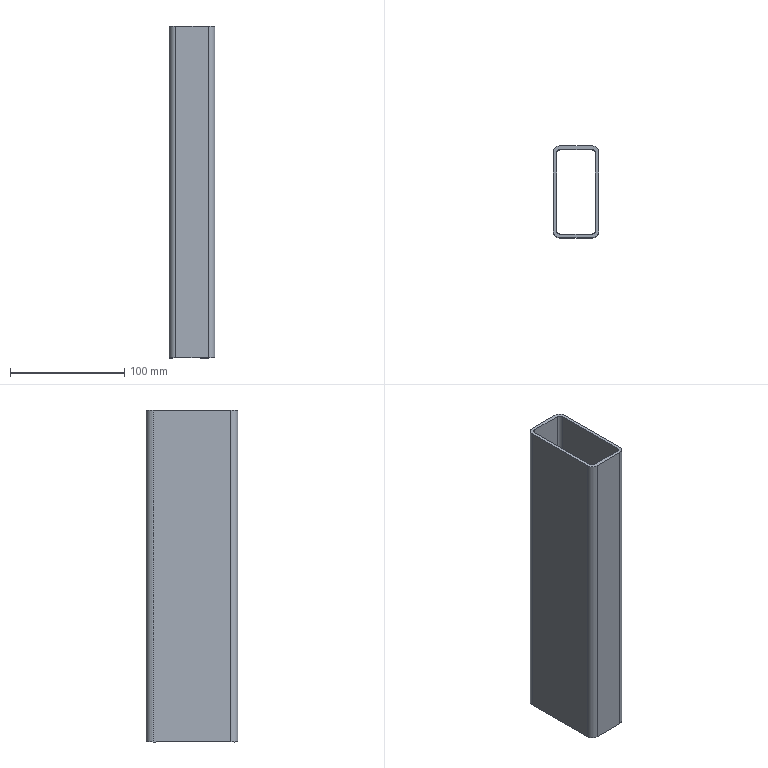Component | SolidWorks | VerticalMovingRectangularTubeWeldment-1_VerticalMovingTube-3 | 1 solid | 18 faces | box 40 x 80 x 290 mm | volume 191639 mm3 | plane 10 | cylinder 8 | commonest cylinder face diameters 12 x4 6 x4 | material Plain Carbon Steel
build123d program:
from build123d import *

# Parameters (mm, degrees)
STRUCTURAL_MEMBER1_DEPTH = 290


with BuildPart() as part:
    # Sketch1 → Structural Member1 (new body)
    with BuildSketch(Plane(origin=(-145, 0, 0), x_dir=(0, 0, -1), z_dir=(1, 0, 0))):
        with BuildLine():
            Line((-14, -40), (14, -40))
            ThreePointArc((14, -40), (18.243, -38.243), (20, -34))
            Line((20, -34), (20, 34))
            ThreePointArc((20, 34), (18.243, 38.243), (14, 40))
            Line((14, 40), (-14, 40))
            ThreePointArc((-14, 40), (-18.243, 38.243), (-20, 34))
            Line((-20, 34), (-20, -34))
            ThreePointArc((-20, -34), (-18.243, -38.243), (-14, -40))
        make_face()
        with BuildLine():
            Line((-14, -37), (14, -37))
            ThreePointArc((14, -37), (16.121, -36.121), (17, -34))
            Line((17, -34), (17, 34))
            ThreePointArc((17, 34), (16.121, 36.121), (14, 37))
            Line((14, 37), (-14, 37))
            ThreePointArc((-14, 37), (-16.121, 36.121), (-17, 34))
            Line((-17, 34), (-17, -34))
            ThreePointArc((-17, -34), (-16.121, -36.121), (-14, -37))
        make_face(mode=Mode.SUBTRACT)
    extrude(amount=STRUCTURAL_MEMBER1_DEPTH)


solid = part.part

# Placed as in the assembly
solid = solid.moved(Location((250, 0, 165), (0, 90, 0)))
STEP:
#1=COLOUR_RGB('',0.7922,0.8196,0.9333);
#2=FILL_AREA_STYLE_COLOUR('',#1);
#3=FILL_AREA_STYLE('',(#2));
#4=SURFACE_STYLE_FILL_AREA(#3);
#5=SURFACE_SIDE_STYLE('',(#4));
#6=SURFACE_STYLE_USAGE(.BOTH.,#5);
#7=PRESENTATION_STYLE_ASSIGNMENT((#6));
#8=CARTESIAN_POINT('',(10.63,1.339,0.7874));
#9=VERTEX_POINT('',#8);
#10=CARTESIAN_POINT('',(10.394,1.575,0.7874));
#11=VERTEX_POINT('',#10);
#12=CARTESIAN_POINT('',(10.394,1.339,0.7874));
#13=DIRECTION('',(-0.,0.,1.));
#14=DIRECTION('',(1.,0.,0.));
#15=AXIS2_PLACEMENT_3D('',#12,#13,#14);
#16=CIRCLE('',#15,0.2362);
#17=EDGE_CURVE('',#9,#11,#16,.T.);
#18=ORIENTED_EDGE('',*,*,#17,.T.);
#19=CARTESIAN_POINT('',(10.394,1.575,12.205));
#20=VERTEX_POINT('',#19);
#21=CARTESIAN_POINT('',(10.394,1.575,12.205));
#22=DIRECTION('',(0.,0.,-1.));
#23=VECTOR('',#22,39.37);
#24=LINE('',#21,#23);
#25=EDGE_CURVE('',#20,#11,#24,.T.);
#26=ORIENTED_EDGE('',*,*,#25,.F.);
#27=CARTESIAN_POINT('',(10.63,1.339,12.205));
#28=VERTEX_POINT('',#27);
#29=CARTESIAN_POINT('',(10.394,1.339,12.205));
#30=DIRECTION('',(-0.,0.,1.));
#31=DIRECTION('',(1.,0.,0.));
#32=AXIS2_PLACEMENT_3D('',#29,#30,#31);
#33=CIRCLE('',#32,0.2362);
#34=EDGE_CURVE('',#28,#20,#33,.T.);
#35=ORIENTED_EDGE('',*,*,#34,.F.);
#36=CARTESIAN_POINT('',(10.63,1.339,12.205));
#37=DIRECTION('',(0.,0.,-1.));
#38=VECTOR('',#37,39.37);
#39=LINE('',#36,#38);
#40=EDGE_CURVE('',#28,#9,#39,.T.);
#41=ORIENTED_EDGE('',*,*,#40,.T.);
#42=EDGE_LOOP('',(#18,#26,#35,#41));
#43=FACE_OUTER_BOUND('',#42,.T.);
#44=CARTESIAN_POINT('',(10.394,1.339,12.205));
#45=DIRECTION('',(0.,0.,-1.));
#46=DIRECTION('',(-1.,0.,0.));
#47=AXIS2_PLACEMENT_3D('',#44,#45,#46);
#48=CYLINDRICAL_SURFACE('',#47,0.2362);
#49=ADVANCED_FACE('',(#43),#48,.T.);
#50=CARTESIAN_POINT('',(9.291,1.575,0.7874));
#51=VERTEX_POINT('',#50);
#52=CARTESIAN_POINT('',(10.394,1.575,0.7874));
#53=DIRECTION('',(-1.,0.,0.));
#54=VECTOR('',#53,39.37);
#55=LINE('',#52,#54);
#56=EDGE_CURVE('',#11,#51,#55,.T.);
#57=ORIENTED_EDGE('',*,*,#56,.T.);
#58=CARTESIAN_POINT('',(9.291,1.575,12.205));
#59=VERTEX_POINT('',#58);
#60=CARTESIAN_POINT('',(9.291,1.575,12.205));
#61=DIRECTION('',(0.,0.,-1.));
#62=VECTOR('',#61,39.37);
#63=LINE('',#60,#62);
#64=EDGE_CURVE('',#59,#51,#63,.T.);
#65=ORIENTED_EDGE('',*,*,#64,.F.);
#66=CARTESIAN_POINT('',(10.394,1.575,12.205));
#67=DIRECTION('',(-1.,0.,0.));
#68=VECTOR('',#67,39.37);
#69=LINE('',#66,#68);
#70=EDGE_CURVE('',#20,#59,#69,.T.);
#71=ORIENTED_EDGE('',*,*,#70,.F.);
#72=ORIENTED_EDGE('',*,*,#25,.T.);
#73=EDGE_LOOP('',(#57,#65,#71,#72));
#74=FACE_OUTER_BOUND('',#73,.T.);
#75=CARTESIAN_POINT('',(10.394,1.575,12.205));
#76=DIRECTION('',(-0.,-1.,0.));
#77=DIRECTION('',(1.,-0.,-0.));
#78=AXIS2_PLACEMENT_3D('',#75,#76,#77);
#79=PLANE('',#78);
#80=ADVANCED_FACE('',(#74),#79,.F.);
#81=CARTESIAN_POINT('',(9.055,1.339,0.7874));
#82=VERTEX_POINT('',#81);
#83=CARTESIAN_POINT('',(9.291,1.339,0.7874));
#84=DIRECTION('',(-0.,0.,1.));
#85=DIRECTION('',(1.,0.,0.));
#86=AXIS2_PLACEMENT_3D('',#83,#84,#85);
#87=CIRCLE('',#86,0.2362);
#88=EDGE_CURVE('',#51,#82,#87,.T.);
#89=ORIENTED_EDGE('',*,*,#88,.T.);
#90=CARTESIAN_POINT('',(9.055,1.339,12.205));
#91=VERTEX_POINT('',#90);
#92=CARTESIAN_POINT('',(9.055,1.339,12.205));
#93=DIRECTION('',(0.,0.,-1.));
#94=VECTOR('',#93,39.37);
#95=LINE('',#92,#94);
#96=EDGE_CURVE('',#91,#82,#95,.T.);
#97=ORIENTED_EDGE('',*,*,#96,.F.);
#98=CARTESIAN_POINT('',(9.291,1.339,12.205));
#99=DIRECTION('',(-0.,0.,1.));
#100=DIRECTION('',(1.,0.,0.));
#101=AXIS2_PLACEMENT_3D('',#98,#99,#100);
#102=CIRCLE('',#101,0.2362);
#103=EDGE_CURVE('',#59,#91,#102,.T.);
#104=ORIENTED_EDGE('',*,*,#103,.F.);
#105=ORIENTED_EDGE('',*,*,#64,.T.);
#106=EDGE_LOOP('',(#89,#97,#104,#105));
#107=FACE_OUTER_BOUND('',#106,.T.);
#108=CARTESIAN_POINT('',(9.291,1.339,12.205));
#109=DIRECTION('',(0.,0.,-1.));
#110=DIRECTION('',(-1.,0.,0.));
#111=AXIS2_PLACEMENT_3D('',#108,#109,#110);
#112=CYLINDRICAL_SURFACE('',#111,0.2362);
#113=ADVANCED_FACE('',(#107),#112,.T.);
#114=CARTESIAN_POINT('',(9.055,-1.339,0.7874));
#115=VERTEX_POINT('',#114);
#116=CARTESIAN_POINT('',(9.055,-1.339,0.7874));
#117=DIRECTION('',(0.,-1.,0.));
#118=VECTOR('',#117,39.37);
#119=LINE('',#116,#118);
#120=EDGE_CURVE('',#82,#115,#119,.T.);
#121=ORIENTED_EDGE('',*,*,#120,.T.);
#122=CARTESIAN_POINT('',(9.055,-1.339,12.205));
#123=VERTEX_POINT('',#122);
#124=CARTESIAN_POINT('',(9.055,-1.339,12.205));
#125=DIRECTION('',(0.,0.,-1.));
#126=VECTOR('',#125,39.37);
#127=LINE('',#124,#126);
#128=EDGE_CURVE('',#123,#115,#127,.T.);
#129=ORIENTED_EDGE('',*,*,#128,.F.);
#130=CARTESIAN_POINT('',(9.055,-1.339,12.205));
#131=DIRECTION('',(0.,-1.,0.));
#132=VECTOR('',#131,39.37);
#133=LINE('',#130,#132);
#134=EDGE_CURVE('',#91,#123,#133,.T.);
#135=ORIENTED_EDGE('',*,*,#134,.F.);
#136=ORIENTED_EDGE('',*,*,#96,.T.);
#137=EDGE_LOOP('',(#121,#129,#135,#136));
#138=FACE_OUTER_BOUND('',#137,.T.);
#139=CARTESIAN_POINT('',(9.055,-1.339,12.205));
#140=DIRECTION('',(1.,-0.,0.));
#141=DIRECTION('',(0.,0.,-1.));
#142=AXIS2_PLACEMENT_3D('',#139,#140,#141);
#143=PLANE('',#142);
#144=ADVANCED_FACE('',(#138),#143,.F.);
#145=CARTESIAN_POINT('',(9.291,-1.575,0.7874));
#146=VERTEX_POINT('',#145);
#147=CARTESIAN_POINT('',(9.291,-1.339,0.7874));
#148=DIRECTION('',(-0.,0.,1.));
#149=DIRECTION('',(1.,0.,0.));
#150=AXIS2_PLACEMENT_3D('',#147,#148,#149);
#151=CIRCLE('',#150,0.2362);
#152=EDGE_CURVE('',#115,#146,#151,.T.);
#153=ORIENTED_EDGE('',*,*,#152,.T.);
#154=CARTESIAN_POINT('',(9.291,-1.575,12.205));
#155=VERTEX_POINT('',#154);
#156=CARTESIAN_POINT('',(9.291,-1.575,12.205));
#157=DIRECTION('',(0.,0.,-1.));
#158=VECTOR('',#157,39.37);
#159=LINE('',#156,#158);
#160=EDGE_CURVE('',#155,#146,#159,.T.);
#161=ORIENTED_EDGE('',*,*,#160,.F.);
#162=CARTESIAN_POINT('',(9.291,-1.339,12.205));
#163=DIRECTION('',(-0.,0.,1.));
#164=DIRECTION('',(1.,0.,0.));
#165=AXIS2_PLACEMENT_3D('',#162,#163,#164);
#166=CIRCLE('',#165,0.2362);
#167=EDGE_CURVE('',#123,#155,#166,.T.);
#168=ORIENTED_EDGE('',*,*,#167,.F.);
#169=ORIENTED_EDGE('',*,*,#128,.T.);
#170=EDGE_LOOP('',(#153,#161,#168,#169));
#171=FACE_OUTER_BOUND('',#170,.T.);
#172=CARTESIAN_POINT('',(9.291,-1.339,12.205));
#173=DIRECTION('',(0.,0.,-1.));
#174=DIRECTION('',(-1.,0.,0.));
#175=AXIS2_PLACEMENT_3D('',#172,#173,#174);
#176=CYLINDRICAL_SURFACE('',#175,0.2362);
#177=ADVANCED_FACE('',(#171),#176,.T.);
#178=CARTESIAN_POINT('',(10.394,-1.575,0.7874));
#179=VERTEX_POINT('',#178);
#180=CARTESIAN_POINT('',(9.291,-1.575,0.7874));
#181=DIRECTION('',(1.,-0.,-0.));
#182=VECTOR('',#181,39.37);
#183=LINE('',#180,#182);
#184=EDGE_CURVE('',#146,#179,#183,.T.);
#185=ORIENTED_EDGE('',*,*,#184,.T.);
#186=CARTESIAN_POINT('',(10.394,-1.575,12.205));
#187=VERTEX_POINT('',#186);
#188=CARTESIAN_POINT('',(10.394,-1.575,12.205));
#189=DIRECTION('',(0.,0.,-1.));
#190=VECTOR('',#189,39.37);
#191=LINE('',#188,#190);
#192=EDGE_CURVE('',#187,#179,#191,.T.);
#193=ORIENTED_EDGE('',*,*,#192,.F.);
#194=CARTESIAN_POINT('',(9.291,-1.575,12.205));
#195=DIRECTION('',(1.,-0.,-0.));
#196=VECTOR('',#195,39.37);
#197=LINE('',#194,#196);
#198=EDGE_CURVE('',#155,#187,#197,.T.);
#199=ORIENTED_EDGE('',*,*,#198,.F.);
#200=ORIENTED_EDGE('',*,*,#160,.T.);
#201=EDGE_LOOP('',(#185,#193,#199,#200));
#202=FACE_OUTER_BOUND('',#201,.T.);
#203=CARTESIAN_POINT('',(9.291,-1.575,12.205));
#204=DIRECTION('',(0.,1.,-0.));
#205=DIRECTION('',(-1.,0.,0.));
#206=AXIS2_PLACEMENT_3D('',#203,#204,#205);
#207=PLANE('',#206);
#208=ADVANCED_FACE('',(#202),#207,.F.);
#209=CARTESIAN_POINT('',(10.63,-1.339,0.7874));
#210=VERTEX_POINT('',#209);
#211=CARTESIAN_POINT('',(10.394,-1.339,0.7874));
#212=DIRECTION('',(-0.,0.,1.));
#213=DIRECTION('',(1.,0.,0.));
#214=AXIS2_PLACEMENT_3D('',#211,#212,#213);
#215=CIRCLE('',#214,0.2362);
#216=EDGE_CURVE('',#179,#210,#215,.T.);
#217=ORIENTED_EDGE('',*,*,#216,.T.);
#218=CARTESIAN_POINT('',(10.63,-1.339,12.205));
#219=VERTEX_POINT('',#218);
#220=CARTESIAN_POINT('',(10.63,-1.339,12.205));
#221=DIRECTION('',(0.,0.,-1.));
#222=VECTOR('',#221,39.37);
#223=LINE('',#220,#222);
#224=EDGE_CURVE('',#219,#210,#223,.T.);
#225=ORIENTED_EDGE('',*,*,#224,.F.);
#226=CARTESIAN_POINT('',(10.394,-1.339,12.205));
#227=DIRECTION('',(-0.,0.,1.));
#228=DIRECTION('',(1.,0.,0.));
#229=AXIS2_PLACEMENT_3D('',#226,#227,#228);
#230=CIRCLE('',#229,0.2362);
#231=EDGE_CURVE('',#187,#219,#230,.T.);
#232=ORIENTED_EDGE('',*,*,#231,.F.);
#233=ORIENTED_EDGE('',*,*,#192,.T.);
#234=EDGE_LOOP('',(#217,#225,#232,#233));
#235=FACE_OUTER_BOUND('',#234,.T.);
#236=CARTESIAN_POINT('',(10.394,-1.339,12.205));
#237=DIRECTION('',(0.,0.,-1.));
#238=DIRECTION('',(-1.,0.,0.));
#239=AXIS2_PLACEMENT_3D('',#236,#237,#238);
#240=CYLINDRICAL_SURFACE('',#239,0.2362);
#241=ADVANCED_FACE('',(#235),#240,.T.);
#242=CARTESIAN_POINT('',(9.291,1.457,0.7874));
#243=VERTEX_POINT('',#242);
#244=CARTESIAN_POINT('',(9.173,1.339,0.7874));
#245=VERTEX_POINT('',#244);
#246=CARTESIAN_POINT('',(9.291,1.339,0.7874));
#247=DIRECTION('',(-0.,0.,1.));
#248=DIRECTION('',(1.,0.,0.));
#249=AXIS2_PLACEMENT_3D('',#246,#247,#248);
#250=CIRCLE('',#249,0.1181);
#251=EDGE_CURVE('',#243,#245,#250,.T.);
#252=ORIENTED_EDGE('',*,*,#251,.F.);
#253=CARTESIAN_POINT('',(9.291,1.457,12.205));
#254=VERTEX_POINT('',#253);
#255=CARTESIAN_POINT('',(9.291,1.457,12.205));
#256=DIRECTION('',(0.,0.,-1.));
#257=VECTOR('',#256,39.37);
#258=LINE('',#255,#257);
#259=EDGE_CURVE('',#254,#243,#258,.T.);
#260=ORIENTED_EDGE('',*,*,#259,.F.);
#261=CARTESIAN_POINT('',(9.173,1.339,12.205));
#262=VERTEX_POINT('',#261);
#263=CARTESIAN_POINT('',(9.291,1.339,12.205));
#264=DIRECTION('',(-0.,0.,1.));
#265=DIRECTION('',(1.,0.,0.));
#266=AXIS2_PLACEMENT_3D('',#263,#264,#265);
#267=CIRCLE('',#266,0.1181);
#268=EDGE_CURVE('',#254,#262,#267,.T.);
#269=ORIENTED_EDGE('',*,*,#268,.T.);
#270=CARTESIAN_POINT('',(9.173,1.339,12.205));
#271=DIRECTION('',(0.,0.,-1.));
#272=VECTOR('',#271,39.37);
#273=LINE('',#270,#272);
#274=EDGE_CURVE('',#262,#245,#273,.T.);
#275=ORIENTED_EDGE('',*,*,#274,.T.);
#276=EDGE_LOOP('',(#252,#260,#269,#275));
#277=FACE_OUTER_BOUND('',#276,.T.);
#278=CARTESIAN_POINT('',(9.291,1.339,12.205));
#279=DIRECTION('',(0.,0.,-1.));
#280=DIRECTION('',(-1.,0.,0.));
#281=AXIS2_PLACEMENT_3D('',#278,#279,#280);
#282=CYLINDRICAL_SURFACE('',#281,0.1181);
#283=ADVANCED_FACE('',(#277),#282,.F.);
#284=CARTESIAN_POINT('',(10.394,1.457,0.7874));
#285=VERTEX_POINT('',#284);
#286=CARTESIAN_POINT('',(10.394,1.457,0.7874));
#287=DIRECTION('',(-1.,0.,0.));
#288=VECTOR('',#287,39.37);
#289=LINE('',#286,#288);
#290=EDGE_CURVE('',#285,#243,#289,.T.);
#291=ORIENTED_EDGE('',*,*,#290,.F.);
#292=CARTESIAN_POINT('',(10.394,1.457,12.205));
#293=VERTEX_POINT('',#292);
#294=CARTESIAN_POINT('',(10.394,1.457,12.205));
#295=DIRECTION('',(0.,0.,-1.));
#296=VECTOR('',#295,39.37);
#297=LINE('',#294,#296);
#298=EDGE_CURVE('',#293,#285,#297,.T.);
#299=ORIENTED_EDGE('',*,*,#298,.F.);
#300=CARTESIAN_POINT('',(10.394,1.457,12.205));
#301=DIRECTION('',(-1.,0.,0.));
#302=VECTOR('',#301,39.37);
#303=LINE('',#300,#302);
#304=EDGE_CURVE('',#293,#254,#303,.T.);
#305=ORIENTED_EDGE('',*,*,#304,.T.);
#306=ORIENTED_EDGE('',*,*,#259,.T.);
#307=EDGE_LOOP('',(#291,#299,#305,#306));
#308=FACE_OUTER_BOUND('',#307,.T.);
#309=CARTESIAN_POINT('',(10.394,1.457,12.205));
#310=DIRECTION('',(-0.,-1.,0.));
#311=DIRECTION('',(1.,-0.,-0.));
#312=AXIS2_PLACEMENT_3D('',#309,#310,#311);
#313=PLANE('',#312);
#314=ADVANCED_FACE('',(#308),#313,.T.);
#315=CARTESIAN_POINT('',(10.512,1.339,0.7874));
#316=VERTEX_POINT('',#315);
#317=CARTESIAN_POINT('',(10.394,1.339,0.7874));
#318=DIRECTION('',(-0.,0.,1.));
#319=DIRECTION('',(1.,0.,0.));
#320=AXIS2_PLACEMENT_3D('',#317,#318,#319);
#321=CIRCLE('',#320,0.1181);
#322=EDGE_CURVE('',#316,#285,#321,.T.);
#323=ORIENTED_EDGE('',*,*,#322,.F.);
#324=CARTESIAN_POINT('',(10.512,1.339,12.205));
#325=VERTEX_POINT('',#324);
#326=CARTESIAN_POINT('',(10.512,1.339,12.205));
#327=DIRECTION('',(0.,0.,-1.));
#328=VECTOR('',#327,39.37);
#329=LINE('',#326,#328);
#330=EDGE_CURVE('',#325,#316,#329,.T.);
#331=ORIENTED_EDGE('',*,*,#330,.F.);
#332=CARTESIAN_POINT('',(10.394,1.339,12.205));
#333=DIRECTION('',(-0.,0.,1.));
#334=DIRECTION('',(1.,0.,0.));
#335=AXIS2_PLACEMENT_3D('',#332,#333,#334);
#336=CIRCLE('',#335,0.1181);
#337=EDGE_CURVE('',#325,#293,#336,.T.);
#338=ORIENTED_EDGE('',*,*,#337,.T.);
#339=ORIENTED_EDGE('',*,*,#298,.T.);
#340=EDGE_LOOP('',(#323,#331,#338,#339));
#341=FACE_OUTER_BOUND('',#340,.T.);
#342=CARTESIAN_POINT('',(10.394,1.339,12.205));
#343=DIRECTION('',(0.,0.,-1.));
#344=DIRECTION('',(-1.,0.,0.));
#345=AXIS2_PLACEMENT_3D('',#342,#343,#344);
#346=CYLINDRICAL_SURFACE('',#345,0.1181);
#347=ADVANCED_FACE('',(#341),#346,.F.);
#348=CARTESIAN_POINT('',(10.512,-1.339,0.7874));
#349=VERTEX_POINT('',#348);
#350=CARTESIAN_POINT('',(10.512,1.339,0.7874));
#351=DIRECTION('',(-0.,1.,0.));
#352=VECTOR('',#351,39.37);
#353=LINE('',#350,#352);
#354=EDGE_CURVE('',#349,#316,#353,.T.);
#355=ORIENTED_EDGE('',*,*,#354,.F.);
#356=CARTESIAN_POINT('',(10.512,-1.339,12.205));
#357=VERTEX_POINT('',#356);
#358=CARTESIAN_POINT('',(10.512,-1.339,12.205));
#359=DIRECTION('',(0.,0.,-1.));
#360=VECTOR('',#359,39.37);
#361=LINE('',#358,#360);
#362=EDGE_CURVE('',#357,#349,#361,.T.);
#363=ORIENTED_EDGE('',*,*,#362,.F.);
#364=CARTESIAN_POINT('',(10.512,1.339,12.205));
#365=DIRECTION('',(-0.,1.,0.));
#366=VECTOR('',#365,39.37);
#367=LINE('',#364,#366);
#368=EDGE_CURVE('',#357,#325,#367,.T.);
#369=ORIENTED_EDGE('',*,*,#368,.T.);
#370=ORIENTED_EDGE('',*,*,#330,.T.);
#371=EDGE_LOOP('',(#355,#363,#369,#370));
#372=FACE_OUTER_BOUND('',#371,.T.);
#373=CARTESIAN_POINT('',(10.512,1.339,12.205));
#374=DIRECTION('',(-1.,0.,-0.));
#375=DIRECTION('',(-0.,0.,1.));
#376=AXIS2_PLACEMENT_3D('',#373,#374,#375);
#377=PLANE('',#376);
#378=ADVANCED_FACE('',(#372),#377,.T.);
#379=CARTESIAN_POINT('',(10.394,-1.457,0.7874));
#380=VERTEX_POINT('',#379);
#381=CARTESIAN_POINT('',(10.394,-1.339,0.7874));
#382=DIRECTION('',(-0.,0.,1.));
#383=DIRECTION('',(1.,0.,0.));
#384=AXIS2_PLACEMENT_3D('',#381,#382,#383);
#385=CIRCLE('',#384,0.1181);
#386=EDGE_CURVE('',#380,#349,#385,.T.);
#387=ORIENTED_EDGE('',*,*,#386,.F.);
#388=CARTESIAN_POINT('',(10.394,-1.457,12.205));
#389=VERTEX_POINT('',#388);
#390=CARTESIAN_POINT('',(10.394,-1.457,12.205));
#391=DIRECTION('',(0.,0.,-1.));
#392=VECTOR('',#391,39.37);
#393=LINE('',#390,#392);
#394=EDGE_CURVE('',#389,#380,#393,.T.);
#395=ORIENTED_EDGE('',*,*,#394,.F.);
#396=CARTESIAN_POINT('',(10.394,-1.339,12.205));
#397=DIRECTION('',(-0.,0.,1.));
#398=DIRECTION('',(1.,0.,0.));
#399=AXIS2_PLACEMENT_3D('',#396,#397,#398);
#400=CIRCLE('',#399,0.1181);
#401=EDGE_CURVE('',#389,#357,#400,.T.);
#402=ORIENTED_EDGE('',*,*,#401,.T.);
#403=ORIENTED_EDGE('',*,*,#362,.T.);
#404=EDGE_LOOP('',(#387,#395,#402,#403));
#405=FACE_OUTER_BOUND('',#404,.T.);
#406=CARTESIAN_POINT('',(10.394,-1.339,12.205));
#407=DIRECTION('',(0.,0.,-1.));
#408=DIRECTION('',(-1.,0.,0.));
#409=AXIS2_PLACEMENT_3D('',#406,#407,#408);
#410=CYLINDRICAL_SURFACE('',#409,0.1181);
#411=ADVANCED_FACE('',(#405),#410,.F.);
#412=CARTESIAN_POINT('',(9.291,-1.457,0.7874));
#413=VERTEX_POINT('',#412);
#414=CARTESIAN_POINT('',(9.291,-1.457,0.7874));
#415=DIRECTION('',(1.,-0.,-0.));
#416=VECTOR('',#415,39.37);
#417=LINE('',#414,#416);
#418=EDGE_CURVE('',#413,#380,#417,.T.);
#419=ORIENTED_EDGE('',*,*,#418,.F.);
#420=CARTESIAN_POINT('',(9.291,-1.457,12.205));
#421=VERTEX_POINT('',#420);
#422=CARTESIAN_POINT('',(9.291,-1.457,12.205));
#423=DIRECTION('',(0.,0.,-1.));
#424=VECTOR('',#423,39.37);
#425=LINE('',#422,#424);
#426=EDGE_CURVE('',#421,#413,#425,.T.);
#427=ORIENTED_EDGE('',*,*,#426,.F.);
#428=CARTESIAN_POINT('',(9.291,-1.457,12.205));
#429=DIRECTION('',(1.,-0.,-0.));
#430=VECTOR('',#429,39.37);
#431=LINE('',#428,#430);
#432=EDGE_CURVE('',#421,#389,#431,.T.);
#433=ORIENTED_EDGE('',*,*,#432,.T.);
#434=ORIENTED_EDGE('',*,*,#394,.T.);
#435=EDGE_LOOP('',(#419,#427,#433,#434));
#436=FACE_OUTER_BOUND('',#435,.T.);
#437=CARTESIAN_POINT('',(9.291,-1.457,12.205));
#438=DIRECTION('',(0.,1.,-0.));
#439=DIRECTION('',(-1.,0.,0.));
#440=AXIS2_PLACEMENT_3D('',#437,#438,#439);
#441=PLANE('',#440);
#442=ADVANCED_FACE('',(#436),#441,.T.);
#443=CARTESIAN_POINT('',(9.173,-1.339,0.7874));
#444=VERTEX_POINT('',#443);
#445=CARTESIAN_POINT('',(9.291,-1.339,0.7874));
#446=DIRECTION('',(-0.,0.,1.));
#447=DIRECTION('',(1.,0.,0.));
#448=AXIS2_PLACEMENT_3D('',#445,#446,#447);
#449=CIRCLE('',#448,0.1181);
#450=EDGE_CURVE('',#444,#413,#449,.T.);
#451=ORIENTED_EDGE('',*,*,#450,.F.);
#452=CARTESIAN_POINT('',(9.173,-1.339,12.205));
#453=VERTEX_POINT('',#452);
#454=CARTESIAN_POINT('',(9.173,-1.339,12.205));
#455=DIRECTION('',(0.,0.,-1.));
#456=VECTOR('',#455,39.37);
#457=LINE('',#454,#456);
#458=EDGE_CURVE('',#453,#444,#457,.T.);
#459=ORIENTED_EDGE('',*,*,#458,.F.);
#460=CARTESIAN_POINT('',(9.291,-1.339,12.205));
#461=DIRECTION('',(-0.,0.,1.));
#462=DIRECTION('',(1.,0.,0.));
#463=AXIS2_PLACEMENT_3D('',#460,#461,#462);
#464=CIRCLE('',#463,0.1181);
#465=EDGE_CURVE('',#453,#421,#464,.T.);
#466=ORIENTED_EDGE('',*,*,#465,.T.);
#467=ORIENTED_EDGE('',*,*,#426,.T.);
#468=EDGE_LOOP('',(#451,#459,#466,#467));
#469=FACE_OUTER_BOUND('',#468,.T.);
#470=CARTESIAN_POINT('',(9.291,-1.339,12.205));
#471=DIRECTION('',(0.,0.,-1.));
#472=DIRECTION('',(-1.,0.,0.));
#473=AXIS2_PLACEMENT_3D('',#470,#471,#472);
#474=CYLINDRICAL_SURFACE('',#473,0.1181);
#475=ADVANCED_FACE('',(#469),#474,.F.);
#476=CARTESIAN_POINT('',(9.173,-1.339,0.7874));
#477=DIRECTION('',(0.,-1.,0.));
#478=VECTOR('',#477,39.37);
#479=LINE('',#476,#478);
#480=EDGE_CURVE('',#245,#444,#479,.T.);
#481=ORIENTED_EDGE('',*,*,#480,.F.);
#482=ORIENTED_EDGE('',*,*,#274,.F.);
#483=CARTESIAN_POINT('',(9.173,-1.339,12.205));
#484=DIRECTION('',(0.,-1.,0.));
#485=VECTOR('',#484,39.37);
#486=LINE('',#483,#485);
#487=EDGE_CURVE('',#262,#453,#486,.T.);
#488=ORIENTED_EDGE('',*,*,#487,.T.);
#489=ORIENTED_EDGE('',*,*,#458,.T.);
#490=EDGE_LOOP('',(#481,#482,#488,#489));
#491=FACE_OUTER_BOUND('',#490,.T.);
#492=CARTESIAN_POINT('',(9.173,-1.339,12.205));
#493=DIRECTION('',(1.,-0.,0.));
#494=DIRECTION('',(0.,0.,-1.));
#495=AXIS2_PLACEMENT_3D('',#492,#493,#494);
#496=PLANE('',#495);
#497=ADVANCED_FACE('',(#491),#496,.T.);
#498=CARTESIAN_POINT('',(10.63,1.339,0.7874));
#499=DIRECTION('',(-0.,1.,0.));
#500=VECTOR('',#499,39.37);
#501=LINE('',#498,#500);
#502=EDGE_CURVE('',#210,#9,#501,.T.);
#503=ORIENTED_EDGE('',*,*,#502,.T.);
#504=ORIENTED_EDGE('',*,*,#40,.F.);
#505=CARTESIAN_POINT('',(10.63,1.339,12.205));
#506=DIRECTION('',(-0.,1.,0.));
#507=VECTOR('',#506,39.37);
#508=LINE('',#505,#507);
#509=EDGE_CURVE('',#219,#28,#508,.T.);
#510=ORIENTED_EDGE('',*,*,#509,.F.);
#511=ORIENTED_EDGE('',*,*,#224,.T.);
#512=EDGE_LOOP('',(#503,#504,#510,#511));
#513=FACE_OUTER_BOUND('',#512,.T.);
#514=CARTESIAN_POINT('',(10.63,1.339,12.205));
#515=DIRECTION('',(-1.,0.,-0.));
#516=DIRECTION('',(-0.,0.,1.));
#517=AXIS2_PLACEMENT_3D('',#514,#515,#516);
#518=PLANE('',#517);
#519=ADVANCED_FACE('',(#513),#518,.F.);
#520=ORIENTED_EDGE('',*,*,#268,.F.);
#521=ORIENTED_EDGE('',*,*,#304,.F.);
#522=ORIENTED_EDGE('',*,*,#337,.F.);
#523=ORIENTED_EDGE('',*,*,#368,.F.);
#524=ORIENTED_EDGE('',*,*,#401,.F.);
#525=ORIENTED_EDGE('',*,*,#432,.F.);
#526=ORIENTED_EDGE('',*,*,#465,.F.);
#527=ORIENTED_EDGE('',*,*,#487,.F.);
#528=EDGE_LOOP('',(#520,#521,#522,#523,#524,#525,#526,#527));
#529=FACE_BOUND('',#528,.T.);
#530=ORIENTED_EDGE('',*,*,#34,.T.);
#531=ORIENTED_EDGE('',*,*,#70,.T.);
#532=ORIENTED_EDGE('',*,*,#103,.T.);
#533=ORIENTED_EDGE('',*,*,#134,.T.);
#534=ORIENTED_EDGE('',*,*,#167,.T.);
#535=ORIENTED_EDGE('',*,*,#198,.T.);
#536=ORIENTED_EDGE('',*,*,#231,.T.);
#537=ORIENTED_EDGE('',*,*,#509,.T.);
#538=EDGE_LOOP('',(#530,#531,#532,#533,#534,#535,#536,#537));
#539=FACE_OUTER_BOUND('',#538,.T.);
#540=CARTESIAN_POINT('',(10.394,1.339,12.205));
#541=DIRECTION('',(0.,-0.,1.));
#542=DIRECTION('',(1.,-0.,-0.));
#543=AXIS2_PLACEMENT_3D('',#540,#541,#542);
#544=PLANE('',#543);
#545=ADVANCED_FACE('',(#529,#539),#544,.T.);
#546=ORIENTED_EDGE('',*,*,#251,.T.);
#547=ORIENTED_EDGE('',*,*,#480,.T.);
#548=ORIENTED_EDGE('',*,*,#450,.T.);
#549=ORIENTED_EDGE('',*,*,#418,.T.);
#550=ORIENTED_EDGE('',*,*,#386,.T.);
#551=ORIENTED_EDGE('',*,*,#354,.T.);
#552=ORIENTED_EDGE('',*,*,#322,.T.);
#553=ORIENTED_EDGE('',*,*,#290,.T.);
#554=EDGE_LOOP('',(#546,#547,#548,#549,#550,#551,#552,#553));
#555=FACE_BOUND('',#554,.T.);
#556=ORIENTED_EDGE('',*,*,#17,.F.);
#557=ORIENTED_EDGE('',*,*,#502,.F.);
#558=ORIENTED_EDGE('',*,*,#216,.F.);
#559=ORIENTED_EDGE('',*,*,#184,.F.);
#560=ORIENTED_EDGE('',*,*,#152,.F.);
#561=ORIENTED_EDGE('',*,*,#120,.F.);
#562=ORIENTED_EDGE('',*,*,#88,.F.);
#563=ORIENTED_EDGE('',*,*,#56,.F.);
#564=EDGE_LOOP('',(#556,#557,#558,#559,#560,#561,#562,#563));
#565=FACE_OUTER_BOUND('',#564,.T.);
#566=CARTESIAN_POINT('',(10.394,1.339,0.7874));
#567=DIRECTION('',(0.,-0.,1.));
#568=DIRECTION('',(1.,-0.,-0.));
#569=AXIS2_PLACEMENT_3D('',#566,#567,#568);
#570=PLANE('',#569);
#571=ADVANCED_FACE('',(#555,#565),#570,.F.);
#572=CLOSED_SHELL('',(#49,#80,#113,#144,#177,#208,#241,#283,#314,#347,#378,#411,#442,#475,#497,#519,#545,#571));
#573=MANIFOLD_SOLID_BREP('',#572);
#574=STYLED_ITEM('',(#7),#573);
#575=(LENGTH_UNIT()NAMED_UNIT(*)SI_UNIT($,.METRE.));
#576=LENGTH_MEASURE_WITH_UNIT(LENGTH_MEASURE(0.0254),#575);
#577=DIMENSIONAL_EXPONENTS(1.,0.,0.,0.,0.,0.,0.);
#578=(CONVERSION_BASED_UNIT('',#576)LENGTH_UNIT()NAMED_UNIT(#577));
#579=UNCERTAINTY_MEASURE_WITH_UNIT(LENGTH_MEASURE(0.00001),#578,'','');
#580=(NAMED_UNIT(*)PLANE_ANGLE_UNIT()SI_UNIT($,.RADIAN.));
#581=(NAMED_UNIT(*)SI_UNIT($,.STERADIAN.)SOLID_ANGLE_UNIT());
#582=(GEOMETRIC_REPRESENTATION_CONTEXT(3)GLOBAL_UNCERTAINTY_ASSIGNED_CONTEXT((#579))GLOBAL_UNIT_ASSIGNED_CONTEXT((#578,#580,#581))REPRESENTATION_CONTEXT('',''));
#583=MECHANICAL_DESIGN_GEOMETRIC_PRESENTATION_REPRESENTATION('',(#574),#582);
#584=PRESENTATION_LAYER_ASSIGNMENT('','',(#574));
#585=CARTESIAN_POINT('',(0.,0.,0.));
#586=DIRECTION('',(0.,0.,1.));
#587=DIRECTION('',(1.,0.,0.));
#588=AXIS2_PLACEMENT_3D('',#585,#586,#587);
#589=(LENGTH_UNIT()NAMED_UNIT(*)SI_UNIT($,.METRE.));
#590=LENGTH_MEASURE_WITH_UNIT(LENGTH_MEASURE(0.0254),#589);
#591=DIMENSIONAL_EXPONENTS(1.,0.,0.,0.,0.,0.,0.);
#592=(CONVERSION_BASED_UNIT('',#590)LENGTH_UNIT()NAMED_UNIT(#591));
#593=UNCERTAINTY_MEASURE_WITH_UNIT(LENGTH_MEASURE(0.00001),#592,'','');
#594=(NAMED_UNIT(*)PLANE_ANGLE_UNIT()SI_UNIT($,.RADIAN.));
#595=(NAMED_UNIT(*)SI_UNIT($,.STERADIAN.)SOLID_ANGLE_UNIT());
#596=(GEOMETRIC_REPRESENTATION_CONTEXT(3)GLOBAL_UNCERTAINTY_ASSIGNED_CONTEXT((#593))GLOBAL_UNIT_ASSIGNED_CONTEXT((#592,#594,#595))REPRESENTATION_CONTEXT('',''));
#597=ADVANCED_BREP_SHAPE_REPRESENTATION('',(#573,#588),#596);